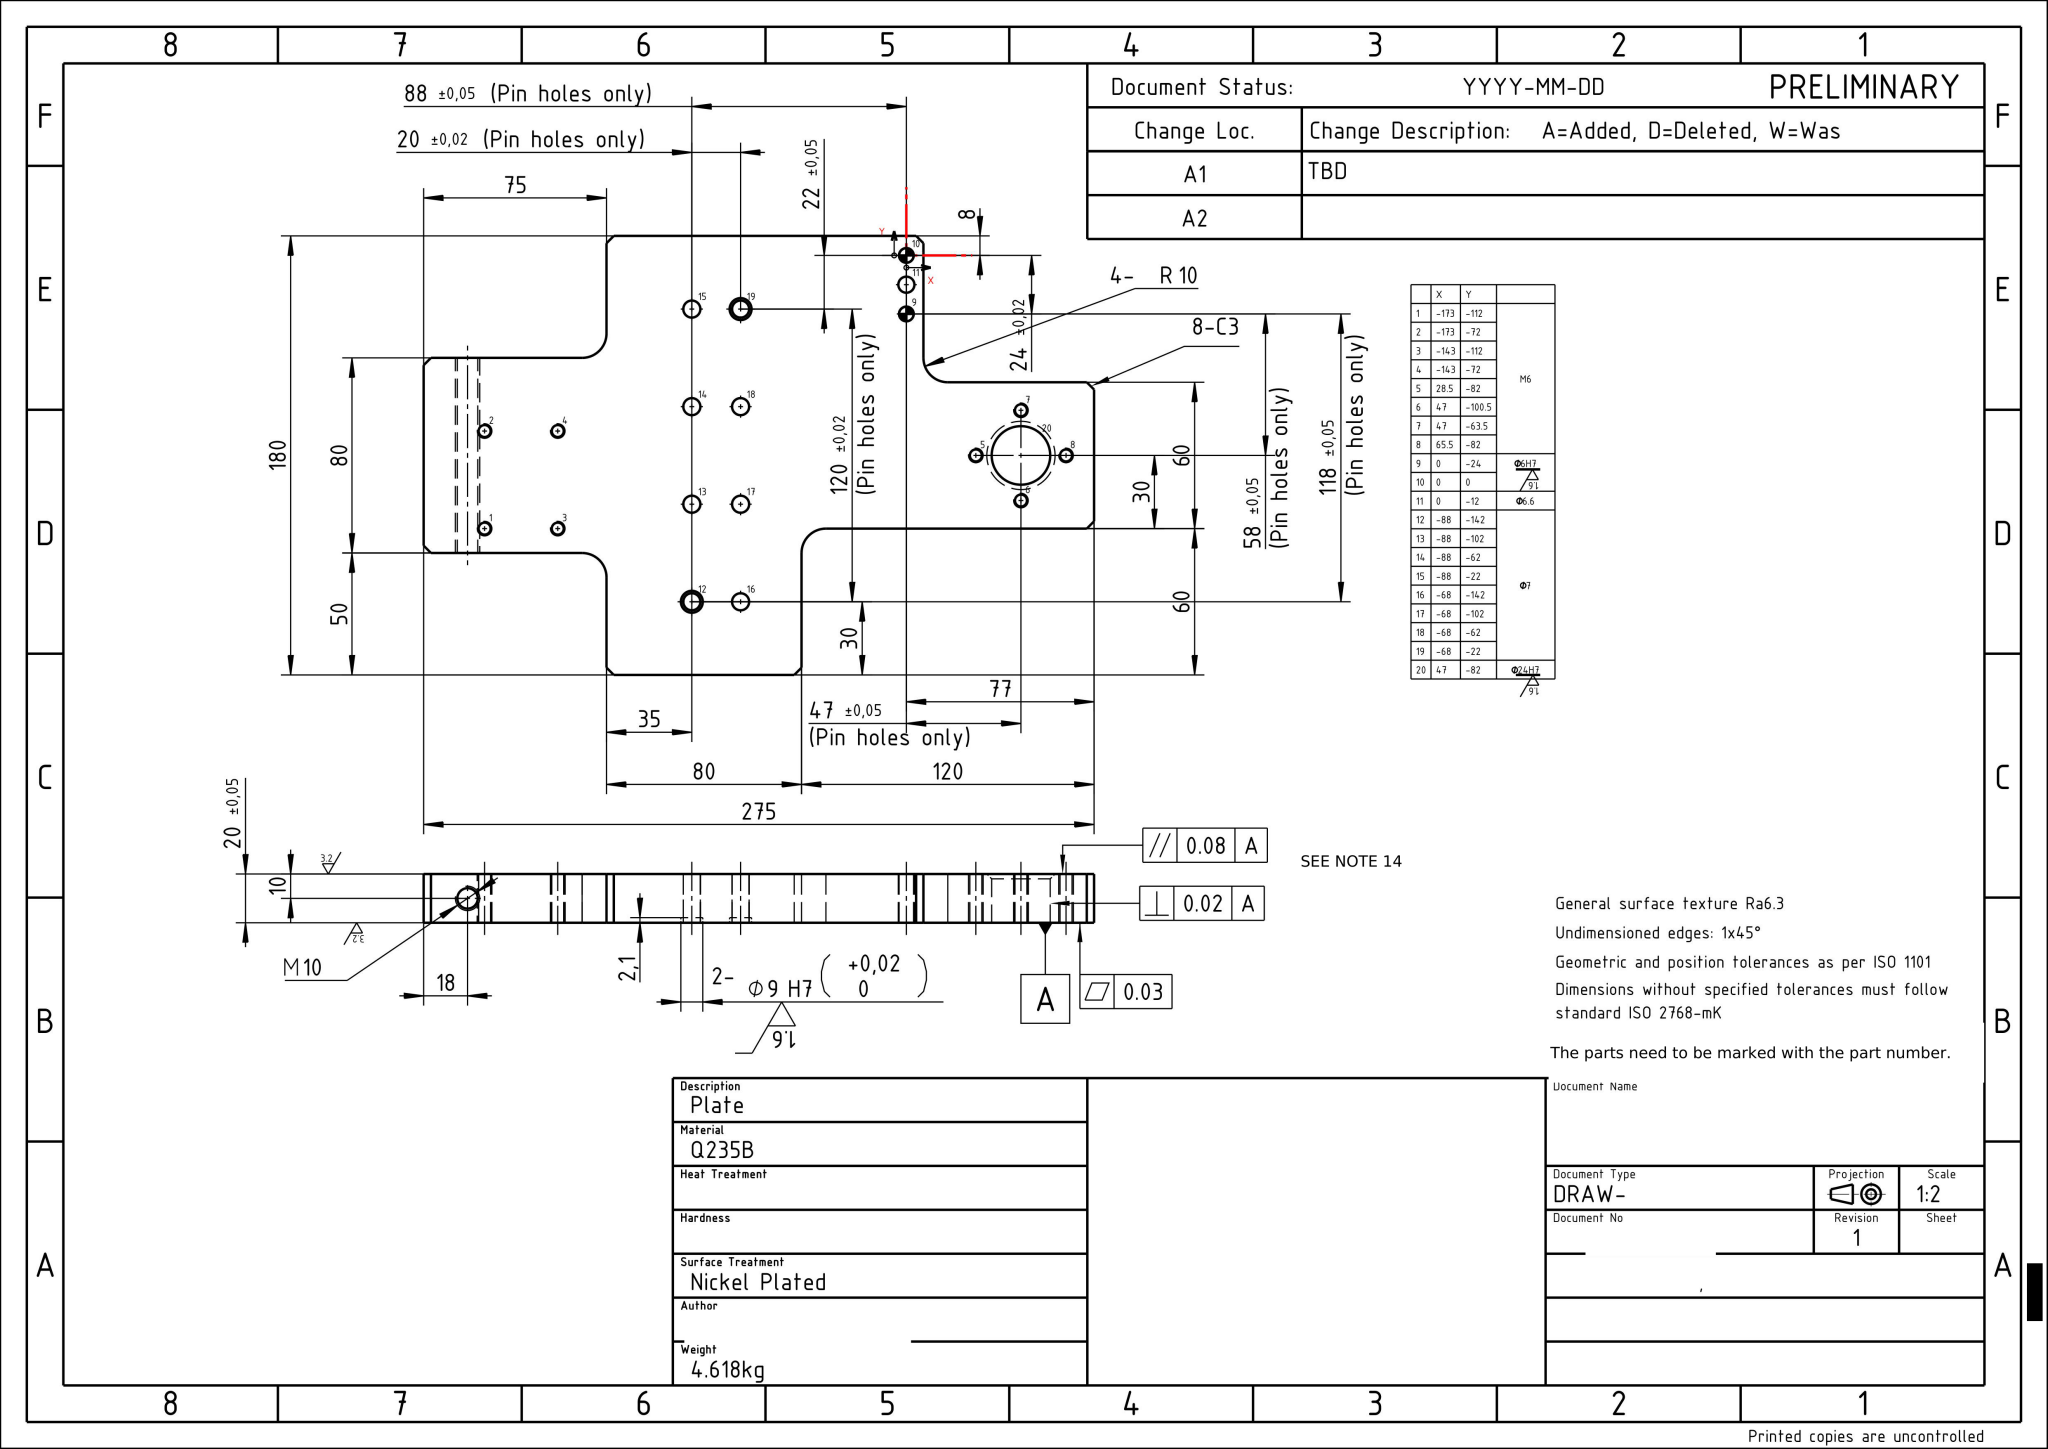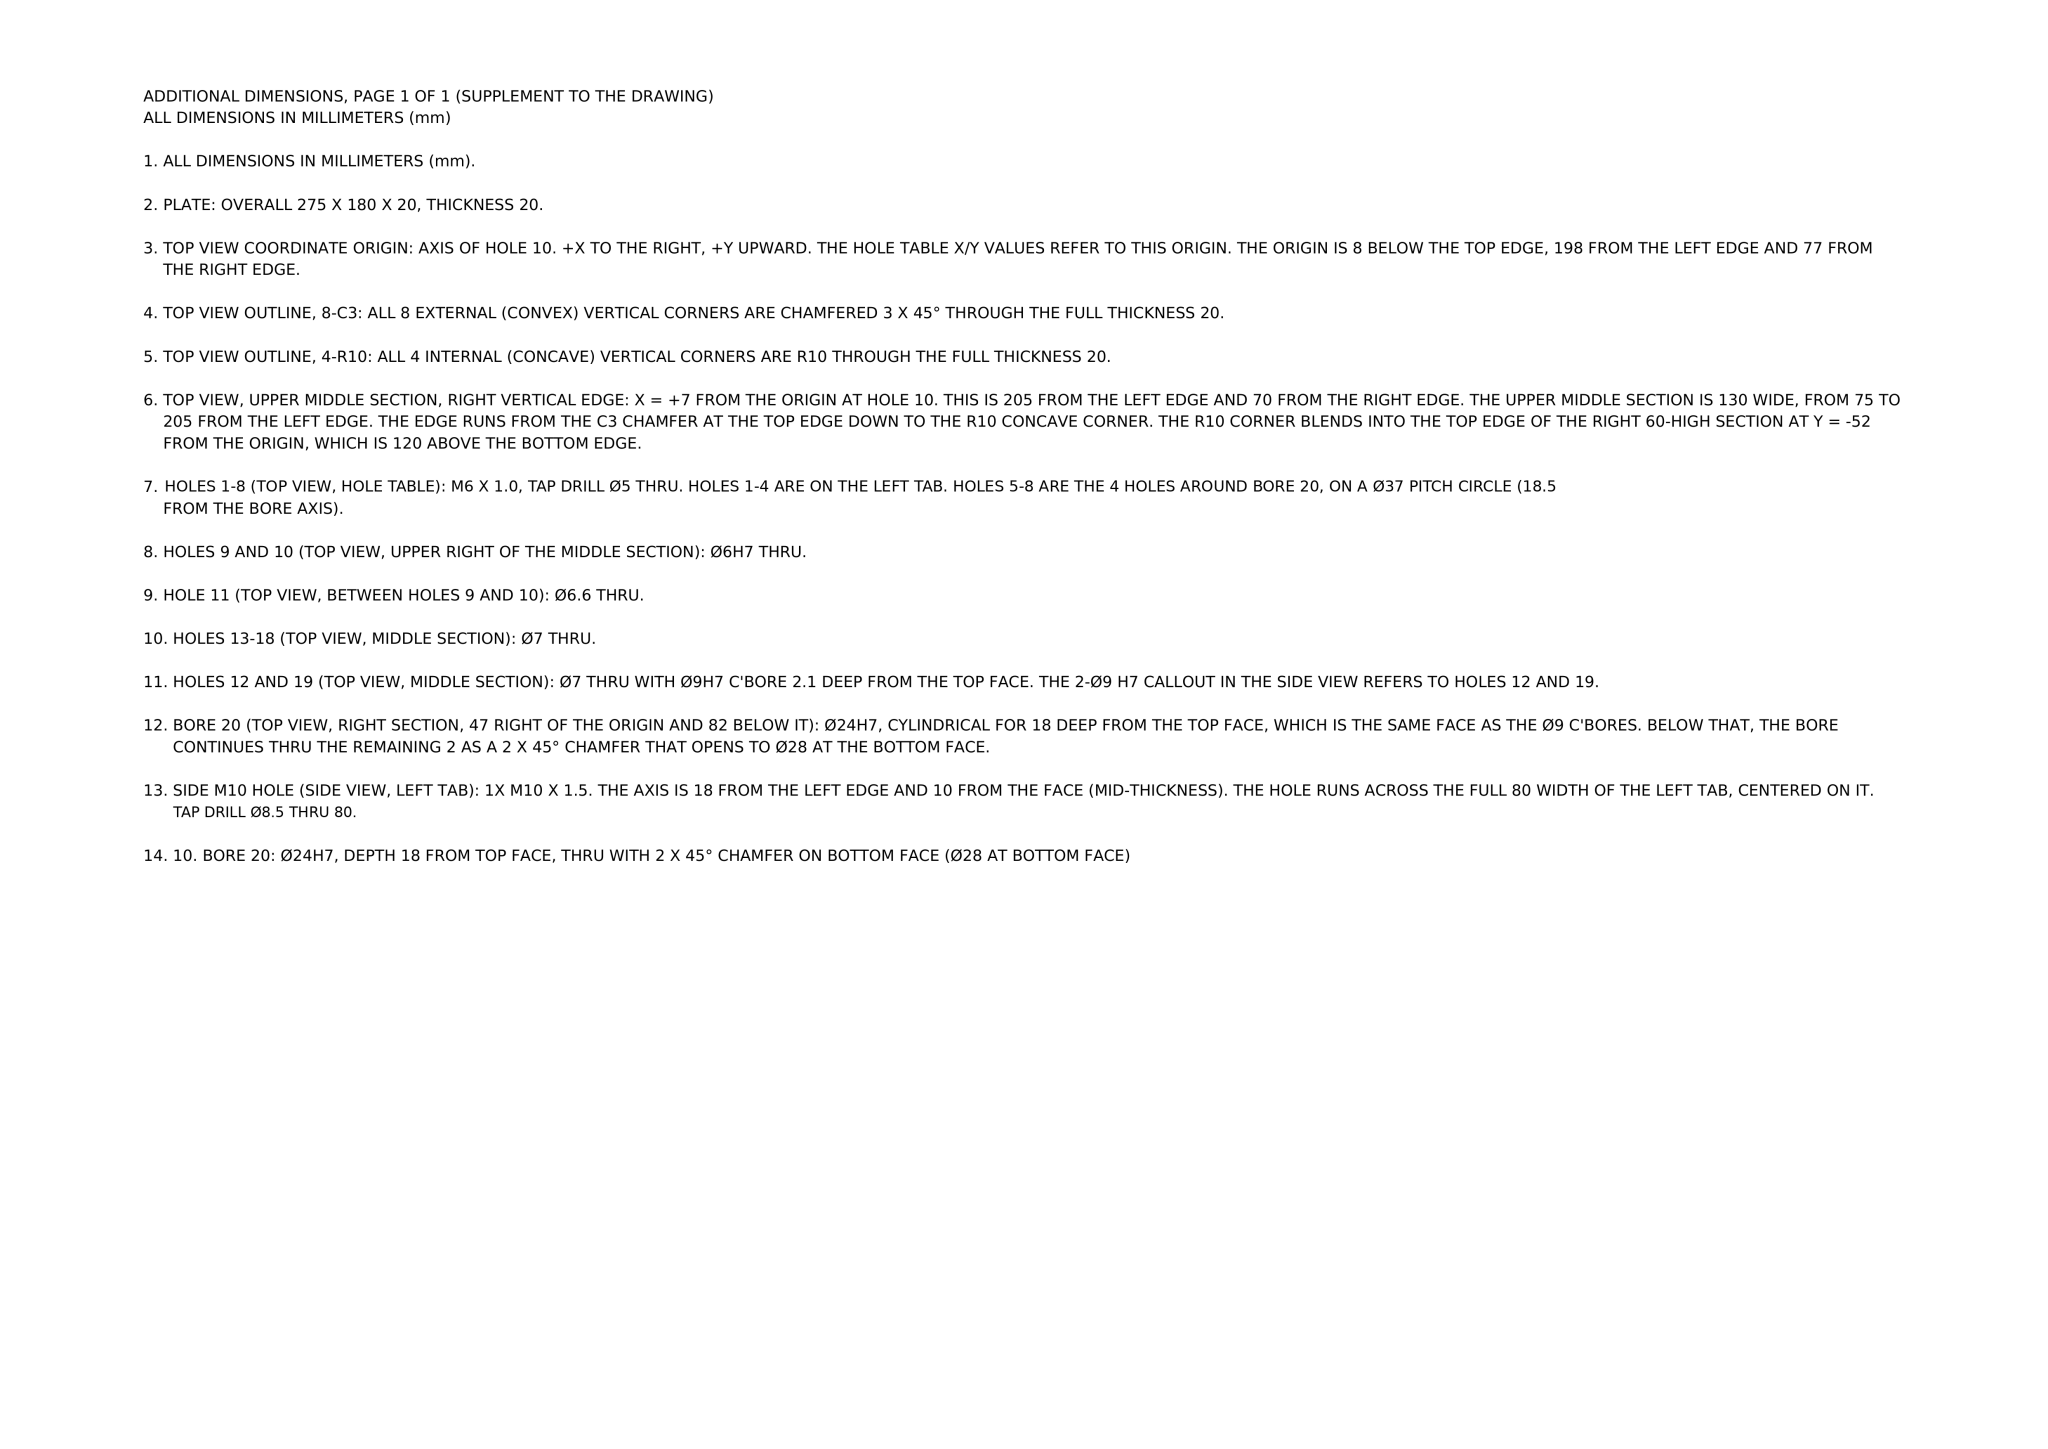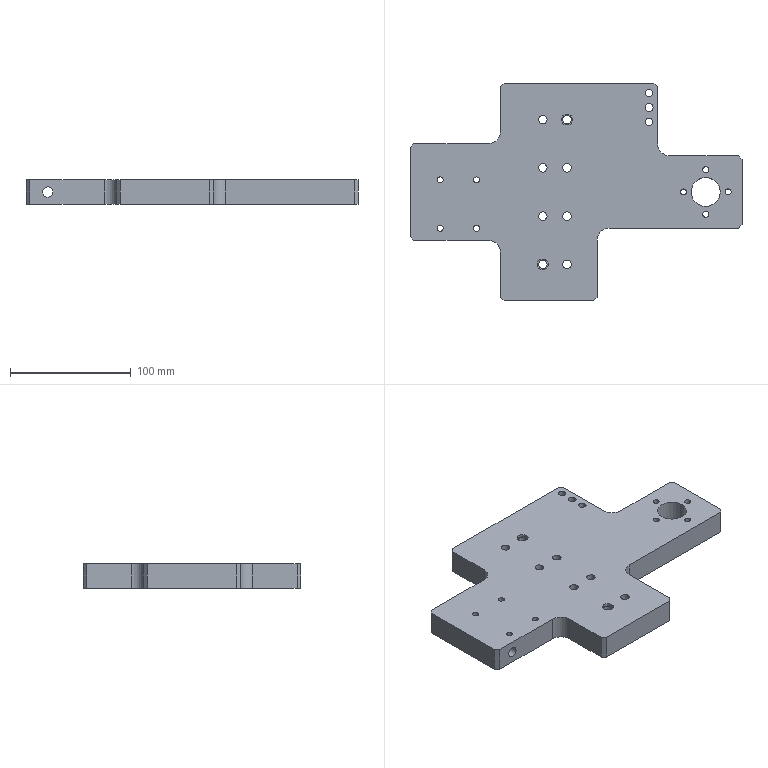Part | NX | mm | 1 solid | 52 faces | box 275 x 180 x 20 mm | volume 588030 mm3 | cylinder 27 | plane 24 | cone 1 | commonest cylinder face diameters 5 x8 7 x8 20 x4 6 x2 9 x2 24 x1 6.6 x1 8.5 x1